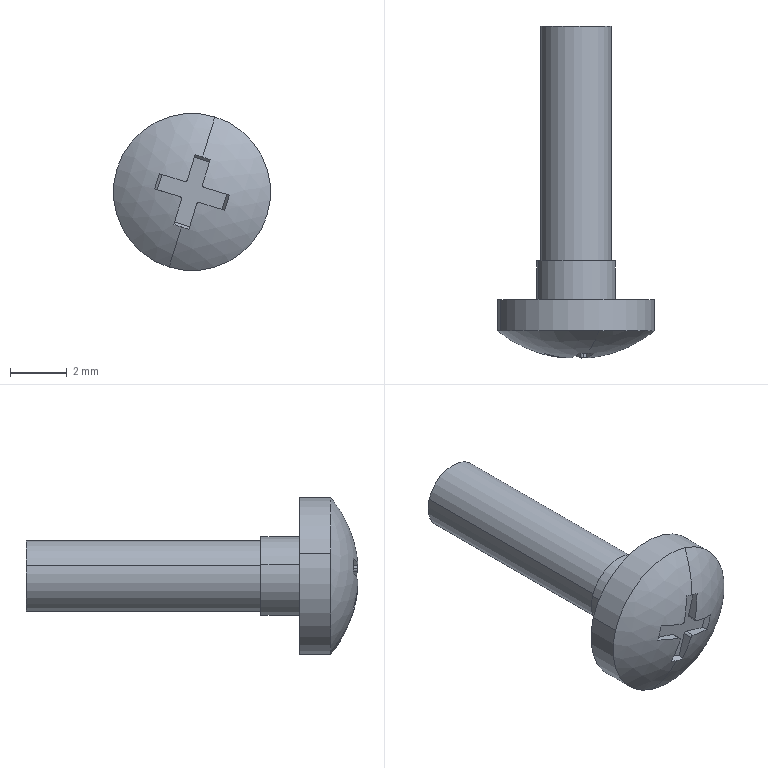Component | SolidWorks | cross recessed small pan head screws gb1-1 | 1 solid | 28 faces | box 5.56 x 11.73 x 5.56 mm | volume 87 mm3 | plane 16 | cylinder 10 | sphere 2 | commonest cylinder face diameters 0.167 x4 2.5 x2 5.556 x2 2.778 x2
STEP:
#1=COLOUR_RGB('',0.7922,0.8196,0.9333);
#2=FILL_AREA_STYLE_COLOUR('',#1);
#3=FILL_AREA_STYLE('',(#2));
#4=SURFACE_STYLE_FILL_AREA(#3);
#5=SURFACE_SIDE_STYLE('',(#4));
#6=SURFACE_STYLE_USAGE(.BOTH.,#5);
#7=PRESENTATION_STYLE_ASSIGNMENT((#6));
#8=CARTESIAN_POINT('',(-0.7465,0.7087,2.14));
#9=VERTEX_POINT('',#8);
#10=CARTESIAN_POINT('',(-0.6523,0.7087,2.112));
#11=VERTEX_POINT('',#10);
#12=CARTESIAN_POINT('',(-0.6994,0.7087,2.126));
#13=DIRECTION('',(0.,1.,0.));
#14=DIRECTION('',(-0.9565,0.,0.2917));
#15=AXIS2_PLACEMENT_3D('',#12,#13,#14);
#16=CIRCLE('',#15,0.04921);
#17=EDGE_CURVE('',#9,#11,#16,.T.);
#18=ORIENTED_EDGE('',*,*,#17,.T.);
#19=CARTESIAN_POINT('',(-0.6523,1.035,2.112));
#20=VERTEX_POINT('',#19);
#21=CARTESIAN_POINT('',(-0.6523,0.7087,2.112));
#22=DIRECTION('',(0.,1.,0.));
#23=VECTOR('',#22,39.37);
#24=LINE('',#21,#23);
#25=EDGE_CURVE('',#11,#20,#24,.T.);
#26=ORIENTED_EDGE('',*,*,#25,.T.);
#27=CARTESIAN_POINT('',(-0.7465,1.035,2.14));
#28=VERTEX_POINT('',#27);
#29=CARTESIAN_POINT('',(-0.6994,1.035,2.126));
#30=DIRECTION('',(0.,1.,0.));
#31=DIRECTION('',(-0.9565,0.,0.2917));
#32=AXIS2_PLACEMENT_3D('',#29,#30,#31);
#33=CIRCLE('',#32,0.04921);
#34=EDGE_CURVE('',#28,#20,#33,.T.);
#35=ORIENTED_EDGE('',*,*,#34,.F.);
#36=CARTESIAN_POINT('',(-0.7465,0.7087,2.14));
#37=DIRECTION('',(0.,1.,0.));
#38=VECTOR('',#37,39.37);
#39=LINE('',#36,#38);
#40=EDGE_CURVE('',#9,#28,#39,.T.);
#41=ORIENTED_EDGE('',*,*,#40,.F.);
#42=EDGE_LOOP('',(#18,#26,#35,#41));
#43=FACE_OUTER_BOUND('',#42,.T.);
#44=CARTESIAN_POINT('',(-0.6994,0.7087,2.126));
#45=DIRECTION('',(0.,1.,0.));
#46=DIRECTION('',(-0.9565,0.,0.2917));
#47=AXIS2_PLACEMENT_3D('',#44,#45,#46);
#48=CYLINDRICAL_SURFACE('',#47,0.04921);
#49=ADVANCED_FACE('',(#43),#48,.T.);
#50=CARTESIAN_POINT('',(-0.6675,0.6111,2.231));
#51=VERTEX_POINT('',#50);
#52=CARTESIAN_POINT('',(-0.5948,0.6111,2.094));
#53=VERTEX_POINT('',#52);
#54=CARTESIAN_POINT('',(-0.6994,0.6111,2.126));
#55=DIRECTION('',(0.,1.,0.));
#56=DIRECTION('',(-0.9565,0.,0.2917));
#57=AXIS2_PLACEMENT_3D('',#54,#55,#56);
#58=CIRCLE('',#57,0.1094);
#59=EDGE_CURVE('',#51,#53,#58,.T.);
#60=ORIENTED_EDGE('',*,*,#59,.T.);
#61=CARTESIAN_POINT('',(-0.5948,0.6548,2.094));
#62=VERTEX_POINT('',#61);
#63=CARTESIAN_POINT('',(-0.5948,0.6221,2.094));
#64=DIRECTION('',(0.,1.,0.));
#65=VECTOR('',#64,39.37);
#66=LINE('',#63,#65);
#67=EDGE_CURVE('',#53,#62,#66,.T.);
#68=ORIENTED_EDGE('',*,*,#67,.T.);
#69=CARTESIAN_POINT('',(-0.804,0.6548,2.158));
#70=VERTEX_POINT('',#69);
#71=CARTESIAN_POINT('',(-0.6994,0.6548,2.126));
#72=DIRECTION('',(0.,1.,0.));
#73=DIRECTION('',(-0.9565,0.,0.2917));
#74=AXIS2_PLACEMENT_3D('',#71,#72,#73);
#75=CIRCLE('',#74,0.1094);
#76=EDGE_CURVE('',#70,#62,#75,.T.);
#77=ORIENTED_EDGE('',*,*,#76,.F.);
#78=CARTESIAN_POINT('',(-0.804,0.6111,2.158));
#79=VERTEX_POINT('',#78);
#80=CARTESIAN_POINT('',(-0.804,0.6221,2.158));
#81=DIRECTION('',(0.,1.,0.));
#82=VECTOR('',#81,39.37);
#83=LINE('',#80,#82);
#84=EDGE_CURVE('',#79,#70,#83,.T.);
#85=ORIENTED_EDGE('',*,*,#84,.F.);
#86=CARTESIAN_POINT('',(-0.6994,0.6111,2.126));
#87=DIRECTION('',(0.,1.,0.));
#88=DIRECTION('',(-0.9565,0.,0.2917));
#89=AXIS2_PLACEMENT_3D('',#86,#87,#88);
#90=CIRCLE('',#89,0.1094);
#91=EDGE_CURVE('',#79,#51,#90,.T.);
#92=ORIENTED_EDGE('',*,*,#91,.T.);
#93=EDGE_LOOP('',(#60,#68,#77,#85,#92));
#94=FACE_OUTER_BOUND('',#93,.T.);
#95=CARTESIAN_POINT('',(-0.6994,0.6221,2.126));
#96=DIRECTION('',(0.,1.,0.));
#97=DIRECTION('',(-0.9565,0.,0.2917));
#98=AXIS2_PLACEMENT_3D('',#95,#96,#97);
#99=CYLINDRICAL_SURFACE('',#98,0.1094);
#100=ADVANCED_FACE('',(#94),#99,.T.);
#101=CARTESIAN_POINT('',(-0.7036,0.5806,2.074));
#102=VERTEX_POINT('',#101);
#103=CARTESIAN_POINT('',(-0.7143,0.5803,2.077));
#104=VERTEX_POINT('',#103);
#105=CARTESIAN_POINT('',(-0.6894,0.7279,2.159));
#106=DIRECTION('',(-0.2527,0.5,-0.8284));
#107=DIRECTION('',(-0.1459,-0.866,-0.4782));
#108=AXIS2_PLACEMENT_3D('',#105,#106,#107);
#109=CIRCLE('',#108,0.1704);
#110=EDGE_CURVE('',#102,#104,#109,.T.);
#111=ORIENTED_EDGE('',*,*,#110,.T.);
#112=CARTESIAN_POINT('',(-0.7313,0.6111,2.021));
#113=VERTEX_POINT('',#112);
#114=CARTESIAN_POINT('',(-0.6994,0.7477,2.126));
#115=DIRECTION('',(0.9565,-0.,-0.2917));
#116=DIRECTION('',(-0.2917,0.,-0.9565));
#117=AXIS2_PLACEMENT_3D('',#114,#115,#116);
#118=CIRCLE('',#117,0.175);
#119=EDGE_CURVE('',#104,#113,#118,.T.);
#120=ORIENTED_EDGE('',*,*,#119,.T.);
#121=CARTESIAN_POINT('',(-0.6994,0.6111,2.126));
#122=DIRECTION('',(0.,1.,0.));
#123=DIRECTION('',(-0.9565,0.,0.2917));
#124=AXIS2_PLACEMENT_3D('',#121,#122,#123);
#125=CIRCLE('',#124,0.1094);
#126=EDGE_CURVE('',#53,#113,#125,.T.);
#127=ORIENTED_EDGE('',*,*,#126,.F.);
#128=ORIENTED_EDGE('',*,*,#59,.F.);
#129=CARTESIAN_POINT('',(-0.6846,0.5803,2.175));
#130=VERTEX_POINT('',#129);
#131=CARTESIAN_POINT('',(-0.6994,0.7477,2.126));
#132=DIRECTION('',(-0.9565,0.,0.2917));
#133=DIRECTION('',(0.2917,0.,0.9565));
#134=AXIS2_PLACEMENT_3D('',#131,#132,#133);
#135=CIRCLE('',#134,0.175);
#136=EDGE_CURVE('',#130,#51,#135,.T.);
#137=ORIENTED_EDGE('',*,*,#136,.F.);
#138=CARTESIAN_POINT('',(-0.6741,0.5806,2.171));
#139=VERTEX_POINT('',#138);
#140=CARTESIAN_POINT('',(-0.7094,0.7279,2.093));
#141=DIRECTION('',(0.2527,0.5,0.8284));
#142=DIRECTION('',(-0.1459,0.866,-0.4782));
#143=AXIS2_PLACEMENT_3D('',#140,#141,#142);
#144=CIRCLE('',#143,0.1704);
#145=EDGE_CURVE('',#130,#139,#144,.T.);
#146=ORIENTED_EDGE('',*,*,#145,.T.);
#147=CARTESIAN_POINT('',(-0.6847,0.5737,2.136));
#148=VERTEX_POINT('',#147);
#149=CARTESIAN_POINT('',(-0.6889,0.7477,2.123));
#150=DIRECTION('',(0.9565,0.,-0.2917));
#151=DIRECTION('',(0.2917,0.,0.9565));
#152=AXIS2_PLACEMENT_3D('',#149,#150,#151);
#153=CIRCLE('',#152,0.1746);
#154=EDGE_CURVE('',#139,#148,#153,.T.);
#155=ORIENTED_EDGE('',*,*,#154,.T.);
#156=CARTESIAN_POINT('',(-0.6825,0.5737,2.132));
#157=VERTEX_POINT('',#156);
#158=CARTESIAN_POINT('',(-0.6847,0.5737,2.136));
#159=CARTESIAN_POINT('',(-0.6848,0.5737,2.136));
#160=CARTESIAN_POINT('',(-0.6848,0.5736,2.136));
#161=CARTESIAN_POINT('',(-0.6848,0.5736,2.135));
#162=CARTESIAN_POINT('',(-0.6848,0.5736,2.135));
#163=CARTESIAN_POINT('',(-0.6847,0.5736,2.135));
#164=CARTESIAN_POINT('',(-0.6846,0.5736,2.134));
#165=CARTESIAN_POINT('',(-0.6845,0.5736,2.134));
#166=CARTESIAN_POINT('',(-0.6843,0.5736,2.134));
#167=CARTESIAN_POINT('',(-0.684,0.5736,2.133));
#168=CARTESIAN_POINT('',(-0.6838,0.5736,2.133));
#169=CARTESIAN_POINT('',(-0.6835,0.5736,2.133));
#170=CARTESIAN_POINT('',(-0.6832,0.5736,2.133));
#171=CARTESIAN_POINT('',(-0.683,0.5736,2.133));
#172=CARTESIAN_POINT('',(-0.6827,0.5737,2.132));
#173=CARTESIAN_POINT('',(-0.6825,0.5737,2.132));
#174=B_SPLINE_CURVE_WITH_KNOTS('',3,(#158,#159,#160,#161,#162,#163,#164,#165,#166,#167,#168,#169,#170,#171,#172,#173),.UNSPECIFIED.,.F.,.F.,(4,3,3,3,3,4),(0.,0.00002794,0.00005589,0.00008373,0.0001115,0.0001303),.UNSPECIFIED.);
#175=EDGE_CURVE('',#148,#157,#174,.T.);
#176=ORIENTED_EDGE('',*,*,#175,.T.);
#177=CARTESIAN_POINT('',(-0.6477,0.5806,2.122));
#178=VERTEX_POINT('',#177);
#179=CARTESIAN_POINT('',(-0.6962,0.7477,2.137));
#180=DIRECTION('',(0.2917,0.,0.9565));
#181=DIRECTION('',(-0.9565,0.,0.2917));
#182=AXIS2_PLACEMENT_3D('',#179,#180,#181);
#183=CIRCLE('',#182,0.1746);
#184=EDGE_CURVE('',#157,#178,#183,.T.);
#185=ORIENTED_EDGE('',*,*,#184,.T.);
#186=CARTESIAN_POINT('',(-0.6542,0.5806,2.101));
#187=VERTEX_POINT('',#186);
#188=CARTESIAN_POINT('',(-0.7323,0.7279,2.136));
#189=DIRECTION('',(0.8284,0.5,-0.2527));
#190=DIRECTION('',(0.4782,-0.866,-0.1459));
#191=AXIS2_PLACEMENT_3D('',#188,#189,#190);
#192=CIRCLE('',#191,0.1704);
#193=EDGE_CURVE('',#178,#187,#192,.T.);
#194=ORIENTED_EDGE('',*,*,#193,.T.);
#195=CARTESIAN_POINT('',(-0.6889,0.5737,2.111));
#196=VERTEX_POINT('',#195);
#197=CARTESIAN_POINT('',(-0.7026,0.7477,2.115));
#198=DIRECTION('',(-0.2917,-0.,-0.9565));
#199=DIRECTION('',(0.9565,-0.,-0.2917));
#200=AXIS2_PLACEMENT_3D('',#197,#198,#199);
#201=CIRCLE('',#200,0.1746);
#202=EDGE_CURVE('',#187,#196,#201,.T.);
#203=ORIENTED_EDGE('',*,*,#202,.T.);
#204=CARTESIAN_POINT('',(-0.693,0.5737,2.109));
#205=VERTEX_POINT('',#204);
#206=CARTESIAN_POINT('',(-0.6889,0.5737,2.111));
#207=CARTESIAN_POINT('',(-0.6893,0.5737,2.111));
#208=CARTESIAN_POINT('',(-0.6897,0.5736,2.111));
#209=CARTESIAN_POINT('',(-0.69,0.5736,2.111));
#210=CARTESIAN_POINT('',(-0.6904,0.5736,2.111));
#211=CARTESIAN_POINT('',(-0.6908,0.5736,2.111));
#212=CARTESIAN_POINT('',(-0.6911,0.5736,2.111));
#213=CARTESIAN_POINT('',(-0.6914,0.5736,2.111));
#214=CARTESIAN_POINT('',(-0.6918,0.5736,2.111));
#215=CARTESIAN_POINT('',(-0.692,0.5736,2.111));
#216=CARTESIAN_POINT('',(-0.6923,0.5736,2.11));
#217=CARTESIAN_POINT('',(-0.6926,0.5736,2.11));
#218=CARTESIAN_POINT('',(-0.6927,0.5736,2.11));
#219=CARTESIAN_POINT('',(-0.6929,0.5736,2.11));
#220=CARTESIAN_POINT('',(-0.693,0.5737,2.109));
#221=CARTESIAN_POINT('',(-0.693,0.5737,2.109));
#222=B_SPLINE_CURVE_WITH_KNOTS('',3,(#206,#207,#208,#209,#210,#211,#212,#213,#214,#215,#216,#217,#218,#219,#220,#221),.UNSPECIFIED.,.F.,.F.,(4,3,3,3,3,4),(0.,0.00002794,0.00005589,0.00008373,0.0001115,0.0001303),.UNSPECIFIED.);
#223=EDGE_CURVE('',#196,#205,#222,.T.);
#224=ORIENTED_EDGE('',*,*,#223,.T.);
#225=CARTESIAN_POINT('',(-0.6889,0.7477,2.123));
#226=DIRECTION('',(0.9565,0.,-0.2917));
#227=DIRECTION('',(0.2917,0.,0.9565));
#228=AXIS2_PLACEMENT_3D('',#225,#226,#227);
#229=CIRCLE('',#228,0.1746);
#230=EDGE_CURVE('',#205,#102,#229,.T.);
#231=ORIENTED_EDGE('',*,*,#230,.T.);
#232=EDGE_LOOP('',(#111,#120,#127,#128,#137,#146,#155,#176,#185,#194,#203,#224,#231));
#233=FACE_OUTER_BOUND('',#232,.T.);
#234=CARTESIAN_POINT('',(-0.6994,0.7477,2.126));
#235=DIRECTION('',(0.9565,-0.,-0.2917));
#236=DIRECTION('',(0.2917,0.,0.9565));
#237=AXIS2_PLACEMENT_3D('',#234,#235,#236);
#238=SPHERICAL_SURFACE('',#237,0.175);
#239=ADVANCED_FACE('',(#233),#238,.T.);
#240=CARTESIAN_POINT('',(-0.7517,0.6548,2.142));
#241=VERTEX_POINT('',#240);
#242=CARTESIAN_POINT('',(-0.6471,0.6548,2.11));
#243=VERTEX_POINT('',#242);
#244=CARTESIAN_POINT('',(-0.6994,0.6548,2.126));
#245=DIRECTION('',(0.,1.,0.));
#246=DIRECTION('',(-0.9565,0.,0.2917));
#247=AXIS2_PLACEMENT_3D('',#244,#245,#246);
#248=CIRCLE('',#247,0.05468);
#249=EDGE_CURVE('',#241,#243,#248,.T.);
#250=ORIENTED_EDGE('',*,*,#249,.T.);
#251=CARTESIAN_POINT('',(-0.6471,0.7087,2.11));
#252=VERTEX_POINT('',#251);
#253=CARTESIAN_POINT('',(-0.6471,0.6221,2.11));
#254=DIRECTION('',(0.,1.,0.));
#255=VECTOR('',#254,39.37);
#256=LINE('',#253,#255);
#257=EDGE_CURVE('',#243,#252,#256,.T.);
#258=ORIENTED_EDGE('',*,*,#257,.T.);
#259=CARTESIAN_POINT('',(-0.7517,0.7087,2.142));
#260=VERTEX_POINT('',#259);
#261=CARTESIAN_POINT('',(-0.6994,0.7087,2.126));
#262=DIRECTION('',(-0.,-1.,0.));
#263=DIRECTION('',(-0.9565,0.,0.2917));
#264=AXIS2_PLACEMENT_3D('',#261,#262,#263);
#265=CIRCLE('',#264,0.05468);
#266=EDGE_CURVE('',#252,#260,#265,.T.);
#267=ORIENTED_EDGE('',*,*,#266,.T.);
#268=CARTESIAN_POINT('',(-0.7517,0.6221,2.142));
#269=DIRECTION('',(0.,1.,0.));
#270=VECTOR('',#269,39.37);
#271=LINE('',#268,#270);
#272=EDGE_CURVE('',#241,#260,#271,.T.);
#273=ORIENTED_EDGE('',*,*,#272,.F.);
#274=EDGE_LOOP('',(#250,#258,#267,#273));
#275=FACE_OUTER_BOUND('',#274,.T.);
#276=CARTESIAN_POINT('',(-0.6994,0.6221,2.126));
#277=DIRECTION('',(0.,1.,0.));
#278=DIRECTION('',(-0.9565,0.,0.2917));
#279=AXIS2_PLACEMENT_3D('',#276,#277,#278);
#280=CYLINDRICAL_SURFACE('',#279,0.05468);
#281=ADVANCED_FACE('',(#275),#280,.T.);
#282=ORIENTED_EDGE('',*,*,#257,.F.);
#283=CARTESIAN_POINT('',(-0.6994,0.6548,2.126));
#284=DIRECTION('',(0.,1.,0.));
#285=DIRECTION('',(-0.9565,0.,0.2917));
#286=AXIS2_PLACEMENT_3D('',#283,#284,#285);
#287=CIRCLE('',#286,0.05468);
#288=EDGE_CURVE('',#243,#241,#287,.T.);
#289=ORIENTED_EDGE('',*,*,#288,.T.);
#290=ORIENTED_EDGE('',*,*,#272,.T.);
#291=CARTESIAN_POINT('',(-0.6994,0.7087,2.126));
#292=DIRECTION('',(-0.,-1.,0.));
#293=DIRECTION('',(-0.9565,0.,0.2917));
#294=AXIS2_PLACEMENT_3D('',#291,#292,#293);
#295=CIRCLE('',#294,0.05468);
#296=EDGE_CURVE('',#260,#252,#295,.T.);
#297=ORIENTED_EDGE('',*,*,#296,.T.);
#298=EDGE_LOOP('',(#282,#289,#290,#297));
#299=FACE_OUTER_BOUND('',#298,.T.);
#300=CARTESIAN_POINT('',(-0.6994,0.6221,2.126));
#301=DIRECTION('',(0.,1.,0.));
#302=DIRECTION('',(-0.9565,0.,0.2917));
#303=AXIS2_PLACEMENT_3D('',#300,#301,#302);
#304=CYLINDRICAL_SURFACE('',#303,0.05468);
#305=ADVANCED_FACE('',(#299),#304,.T.);
#306=ORIENTED_EDGE('',*,*,#119,.F.);
#307=CARTESIAN_POINT('',(-0.7248,0.5806,2.081));
#308=VERTEX_POINT('',#307);
#309=CARTESIAN_POINT('',(-0.6894,0.7279,2.159));
#310=DIRECTION('',(-0.2527,0.5,-0.8284));
#311=DIRECTION('',(-0.1459,-0.866,-0.4782));
#312=AXIS2_PLACEMENT_3D('',#309,#310,#311);
#313=CIRCLE('',#312,0.1704);
#314=EDGE_CURVE('',#104,#308,#313,.T.);
#315=ORIENTED_EDGE('',*,*,#314,.T.);
#316=CARTESIAN_POINT('',(-0.7142,0.5737,2.116));
#317=VERTEX_POINT('',#316);
#318=CARTESIAN_POINT('',(-0.71,0.7477,2.129));
#319=DIRECTION('',(-0.9565,-0.,0.2917));
#320=DIRECTION('',(0.,1.,0.));
#321=AXIS2_PLACEMENT_3D('',#318,#319,#320);
#322=CIRCLE('',#321,0.1746);
#323=EDGE_CURVE('',#308,#317,#322,.T.);
#324=ORIENTED_EDGE('',*,*,#323,.T.);
#325=CARTESIAN_POINT('',(-0.7163,0.5737,2.12));
#326=VERTEX_POINT('',#325);
#327=CARTESIAN_POINT('',(-0.7142,0.5737,2.116));
#328=CARTESIAN_POINT('',(-0.7141,0.5737,2.116));
#329=CARTESIAN_POINT('',(-0.714,0.5736,2.116));
#330=CARTESIAN_POINT('',(-0.714,0.5736,2.117));
#331=CARTESIAN_POINT('',(-0.714,0.5736,2.117));
#332=CARTESIAN_POINT('',(-0.7141,0.5736,2.117));
#333=CARTESIAN_POINT('',(-0.7143,0.5736,2.118));
#334=CARTESIAN_POINT('',(-0.7144,0.5736,2.118));
#335=CARTESIAN_POINT('',(-0.7146,0.5736,2.118));
#336=CARTESIAN_POINT('',(-0.7148,0.5736,2.119));
#337=CARTESIAN_POINT('',(-0.7151,0.5736,2.119));
#338=CARTESIAN_POINT('',(-0.7153,0.5736,2.119));
#339=CARTESIAN_POINT('',(-0.7157,0.5736,2.119));
#340=CARTESIAN_POINT('',(-0.7159,0.5736,2.119));
#341=CARTESIAN_POINT('',(-0.7161,0.5737,2.12));
#342=CARTESIAN_POINT('',(-0.7163,0.5737,2.12));
#343=B_SPLINE_CURVE_WITH_KNOTS('',3,(#327,#328,#329,#330,#331,#332,#333,#334,#335,#336,#337,#338,#339,#340,#341,#342),.UNSPECIFIED.,.F.,.F.,(4,3,3,3,3,4),(0.,0.00002794,0.00005589,0.00008373,0.0001115,0.0001303),.UNSPECIFIED.);
#344=EDGE_CURVE('',#317,#326,#343,.T.);
#345=ORIENTED_EDGE('',*,*,#344,.T.);
#346=CARTESIAN_POINT('',(-0.7511,0.5806,2.13));
#347=VERTEX_POINT('',#346);
#348=CARTESIAN_POINT('',(-0.7026,0.7477,2.115));
#349=DIRECTION('',(-0.2917,0.,-0.9565));
#350=DIRECTION('',(0.9565,0.,-0.2917));
#351=AXIS2_PLACEMENT_3D('',#348,#349,#350);
#352=CIRCLE('',#351,0.1746);
#353=EDGE_CURVE('',#326,#347,#352,.T.);
#354=ORIENTED_EDGE('',*,*,#353,.T.);
#355=CARTESIAN_POINT('',(-0.7447,0.5806,2.151));
#356=VERTEX_POINT('',#355);
#357=CARTESIAN_POINT('',(-0.6666,0.7279,2.116));
#358=DIRECTION('',(-0.8284,0.5,0.2527));
#359=DIRECTION('',(0.4782,0.866,-0.1459));
#360=AXIS2_PLACEMENT_3D('',#357,#358,#359);
#361=CIRCLE('',#360,0.1704);
#362=EDGE_CURVE('',#347,#356,#361,.T.);
#363=ORIENTED_EDGE('',*,*,#362,.T.);
#364=CARTESIAN_POINT('',(-0.7099,0.5737,2.141));
#365=VERTEX_POINT('',#364);
#366=CARTESIAN_POINT('',(-0.6962,0.7477,2.137));
#367=DIRECTION('',(0.2917,0.,0.9565));
#368=DIRECTION('',(-0.9565,-0.,0.2917));
#369=AXIS2_PLACEMENT_3D('',#366,#367,#368);
#370=CIRCLE('',#369,0.1746);
#371=EDGE_CURVE('',#356,#365,#370,.T.);
#372=ORIENTED_EDGE('',*,*,#371,.T.);
#373=CARTESIAN_POINT('',(-0.7058,0.5737,2.143));
#374=VERTEX_POINT('',#373);
#375=CARTESIAN_POINT('',(-0.7099,0.5737,2.141));
#376=CARTESIAN_POINT('',(-0.7096,0.5737,2.141));
#377=CARTESIAN_POINT('',(-0.7092,0.5736,2.141));
#378=CARTESIAN_POINT('',(-0.7088,0.5736,2.141));
#379=CARTESIAN_POINT('',(-0.7084,0.5736,2.141));
#380=CARTESIAN_POINT('',(-0.7081,0.5736,2.141));
#381=CARTESIAN_POINT('',(-0.7077,0.5736,2.141));
#382=CARTESIAN_POINT('',(-0.7074,0.5736,2.141));
#383=CARTESIAN_POINT('',(-0.7071,0.5736,2.141));
#384=CARTESIAN_POINT('',(-0.7068,0.5736,2.141));
#385=CARTESIAN_POINT('',(-0.7065,0.5736,2.142));
#386=CARTESIAN_POINT('',(-0.7063,0.5736,2.142));
#387=CARTESIAN_POINT('',(-0.7061,0.5736,2.142));
#388=CARTESIAN_POINT('',(-0.706,0.5736,2.142));
#389=CARTESIAN_POINT('',(-0.7059,0.5737,2.143));
#390=CARTESIAN_POINT('',(-0.7058,0.5737,2.143));
#391=B_SPLINE_CURVE_WITH_KNOTS('',3,(#375,#376,#377,#378,#379,#380,#381,#382,#383,#384,#385,#386,#387,#388,#389,#390),.UNSPECIFIED.,.F.,.F.,(4,3,3,3,3,4),(0.,0.00002794,0.00005589,0.00008373,0.0001115,0.0001303),.UNSPECIFIED.);
#392=EDGE_CURVE('',#365,#374,#391,.T.);
#393=ORIENTED_EDGE('',*,*,#392,.T.);
#394=CARTESIAN_POINT('',(-0.6952,0.5806,2.178));
#395=VERTEX_POINT('',#394);
#396=CARTESIAN_POINT('',(-0.71,0.7477,2.129));
#397=DIRECTION('',(-0.9565,-0.,0.2917));
#398=DIRECTION('',(0.,1.,0.));
#399=AXIS2_PLACEMENT_3D('',#396,#397,#398);
#400=CIRCLE('',#399,0.1746);
#401=EDGE_CURVE('',#374,#395,#400,.T.);
#402=ORIENTED_EDGE('',*,*,#401,.T.);
#403=CARTESIAN_POINT('',(-0.7094,0.7279,2.093));
#404=DIRECTION('',(0.2527,0.5,0.8284));
#405=DIRECTION('',(-0.1459,0.866,-0.4782));
#406=AXIS2_PLACEMENT_3D('',#403,#404,#405);
#407=CIRCLE('',#406,0.1704);
#408=EDGE_CURVE('',#395,#130,#407,.T.);
#409=ORIENTED_EDGE('',*,*,#408,.T.);
#410=ORIENTED_EDGE('',*,*,#136,.T.);
#411=ORIENTED_EDGE('',*,*,#91,.F.);
#412=CARTESIAN_POINT('',(-0.6994,0.6111,2.126));
#413=DIRECTION('',(0.,1.,0.));
#414=DIRECTION('',(-0.9565,0.,0.2917));
#415=AXIS2_PLACEMENT_3D('',#412,#413,#414);
#416=CIRCLE('',#415,0.1094);
#417=EDGE_CURVE('',#113,#79,#416,.T.);
#418=ORIENTED_EDGE('',*,*,#417,.F.);
#419=EDGE_LOOP('',(#306,#315,#324,#345,#354,#363,#372,#393,#402,#409,#410,#411,#418));
#420=FACE_OUTER_BOUND('',#419,.T.);
#421=CARTESIAN_POINT('',(-0.6994,0.7477,2.126));
#422=DIRECTION('',(0.9565,-0.,-0.2917));
#423=DIRECTION('',(0.2917,0.,0.9565));
#424=AXIS2_PLACEMENT_3D('',#421,#422,#423);
#425=SPHERICAL_SURFACE('',#424,0.175);
#426=ADVANCED_FACE('',(#420),#425,.T.);
#427=ORIENTED_EDGE('',*,*,#76,.T.);
#428=CARTESIAN_POINT('',(-0.6994,0.6548,2.126));
#429=DIRECTION('',(0.,1.,0.));
#430=DIRECTION('',(-0.9565,0.,0.2917));
#431=AXIS2_PLACEMENT_3D('',#428,#429,#430);
#432=CIRCLE('',#431,0.1094);
#433=EDGE_CURVE('',#62,#70,#432,.T.);
#434=ORIENTED_EDGE('',*,*,#433,.T.);
#435=EDGE_LOOP('',(#427,#434));
#436=FACE_OUTER_BOUND('',#435,.T.);
#437=ORIENTED_EDGE('',*,*,#249,.F.);
#438=ORIENTED_EDGE('',*,*,#288,.F.);
#439=EDGE_LOOP('',(#437,#438));
#440=FACE_BOUND('',#439,.T.);
#441=CARTESIAN_POINT('',(-0.6816,0.6548,2.185));
#442=DIRECTION('',(0.,1.,0.));
#443=DIRECTION('',(-0.9565,-0.,0.2917));
#444=AXIS2_PLACEMENT_3D('',#441,#442,#443);
#445=PLANE('',#444);
#446=ADVANCED_FACE('',(#436,#440),#445,.T.);
#447=ORIENTED_EDGE('',*,*,#67,.F.);
#448=ORIENTED_EDGE('',*,*,#126,.T.);
#449=ORIENTED_EDGE('',*,*,#417,.T.);
#450=ORIENTED_EDGE('',*,*,#84,.T.);
#451=ORIENTED_EDGE('',*,*,#433,.F.);
#452=EDGE_LOOP('',(#447,#448,#449,#450,#451));
#453=FACE_OUTER_BOUND('',#452,.T.);
#454=CARTESIAN_POINT('',(-0.6994,0.6221,2.126));
#455=DIRECTION('',(0.,1.,0.));
#456=DIRECTION('',(-0.9565,0.,0.2917));
#457=AXIS2_PLACEMENT_3D('',#454,#455,#456);
#458=CYLINDRICAL_SURFACE('',#457,0.1094);
#459=ADVANCED_FACE('',(#453),#458,.T.);
#460=ORIENTED_EDGE('',*,*,#184,.F.);
#461=CARTESIAN_POINT('',(-0.6825,0.587,2.132));
#462=VERTEX_POINT('',#461);
#463=CARTESIAN_POINT('',(-0.6825,0.587,2.132));
#464=DIRECTION('',(0.,1.,0.));
#465=VECTOR('',#464,39.37);
#466=LINE('',#463,#465);
#467=EDGE_CURVE('',#157,#462,#466,.T.);
#468=ORIENTED_EDGE('',*,*,#467,.T.);
#469=CARTESIAN_POINT('',(-0.6512,0.587,2.123));
#470=VERTEX_POINT('',#469);
#471=CARTESIAN_POINT('',(-0.6856,0.587,2.133));
#472=DIRECTION('',(0.9565,0.,-0.2917));
#473=VECTOR('',#472,39.37);
#474=LINE('',#471,#473);
#475=EDGE_CURVE('',#462,#470,#474,.T.);
#476=ORIENTED_EDGE('',*,*,#475,.T.);
#477=CARTESIAN_POINT('',(-0.6434,0.5727,2.12));
#478=DIRECTION('',(0.4782,-0.866,-0.1459));
#479=VECTOR('',#478,39.37);
#480=LINE('',#477,#479);
#481=EDGE_CURVE('',#470,#178,#480,.T.);
#482=ORIENTED_EDGE('',*,*,#481,.T.);
#483=EDGE_LOOP('',(#460,#468,#476,#482));
#484=FACE_OUTER_BOUND('',#483,.T.);
#485=CARTESIAN_POINT('',(-0.6856,0.587,2.133));
#486=DIRECTION('',(-0.2917,-0.,-0.9565));
#487=DIRECTION('',(-0.9565,-0.,0.2917));
#488=AXIS2_PLACEMENT_3D('',#485,#486,#487);
#489=PLANE('',#488);
#490=ADVANCED_FACE('',(#484),#489,.T.);
#491=ORIENTED_EDGE('',*,*,#481,.F.);
#492=CARTESIAN_POINT('',(-0.6577,0.587,2.102));
#493=VERTEX_POINT('',#492);
#494=CARTESIAN_POINT('',(-0.6544,0.587,2.112));
#495=DIRECTION('',(-0.2917,0.,-0.9565));
#496=VECTOR('',#495,39.37);
#497=LINE('',#494,#496);
#498=EDGE_CURVE('',#470,#493,#497,.T.);
#499=ORIENTED_EDGE('',*,*,#498,.T.);
#500=CARTESIAN_POINT('',(-0.6663,0.6025,2.104));
#501=DIRECTION('',(0.4782,-0.866,-0.1459));
#502=VECTOR('',#501,39.37);
#503=LINE('',#500,#502);
#504=EDGE_CURVE('',#493,#187,#503,.T.);
#505=ORIENTED_EDGE('',*,*,#504,.T.);
#506=ORIENTED_EDGE('',*,*,#193,.F.);
#507=EDGE_LOOP('',(#491,#499,#505,#506));
#508=FACE_OUTER_BOUND('',#507,.T.);
#509=CARTESIAN_POINT('',(-0.6466,0.5727,2.11));
#510=DIRECTION('',(-0.8284,-0.5,0.2527));
#511=DIRECTION('',(0.4782,-0.866,-0.1459));
#512=AXIS2_PLACEMENT_3D('',#509,#510,#511);
#513=PLANE('',#512);
#514=ADVANCED_FACE('',(#508),#513,.T.);
#515=CARTESIAN_POINT('',(-0.6889,0.587,2.111));
#516=VERTEX_POINT('',#515);
#517=CARTESIAN_POINT('',(-0.6921,0.587,2.112));
#518=DIRECTION('',(-0.9565,-0.,0.2917));
#519=VECTOR('',#518,39.37);
#520=LINE('',#517,#519);
#521=EDGE_CURVE('',#493,#516,#520,.T.);
#522=ORIENTED_EDGE('',*,*,#521,.T.);
#523=CARTESIAN_POINT('',(-0.6889,0.587,2.111));
#524=DIRECTION('',(-0.,-1.,0.));
#525=VECTOR('',#524,39.37);
#526=LINE('',#523,#525);
#527=EDGE_CURVE('',#516,#196,#526,.T.);
#528=ORIENTED_EDGE('',*,*,#527,.T.);
#529=ORIENTED_EDGE('',*,*,#202,.F.);
#530=ORIENTED_EDGE('',*,*,#504,.F.);
#531=EDGE_LOOP('',(#522,#528,#529,#530));
#532=FACE_OUTER_BOUND('',#531,.T.);
#533=CARTESIAN_POINT('',(-0.6921,0.587,2.112));
#534=DIRECTION('',(0.2917,0.,0.9565));
#535=DIRECTION('',(0.9565,0.,-0.2917));
#536=AXIS2_PLACEMENT_3D('',#533,#534,#535);
#537=PLANE('',#536);
#538=ADVANCED_FACE('',(#532),#537,.T.);
#539=ORIENTED_EDGE('',*,*,#230,.F.);
#540=CARTESIAN_POINT('',(-0.693,0.587,2.109));
#541=VERTEX_POINT('',#540);
#542=CARTESIAN_POINT('',(-0.693,0.587,2.109));
#543=DIRECTION('',(0.,1.,0.));
#544=VECTOR('',#543,39.37);
#545=LINE('',#542,#544);
#546=EDGE_CURVE('',#205,#541,#545,.T.);
#547=ORIENTED_EDGE('',*,*,#546,.T.);
#548=CARTESIAN_POINT('',(-0.7026,0.587,2.078));
#549=VERTEX_POINT('',#548);
#550=CARTESIAN_POINT('',(-0.6921,0.587,2.112));
#551=DIRECTION('',(-0.2917,-0.,-0.9565));
#552=VECTOR('',#551,39.37);
#553=LINE('',#550,#552);
#554=EDGE_CURVE('',#541,#549,#553,.T.);
#555=ORIENTED_EDGE('',*,*,#554,.T.);
#556=CARTESIAN_POINT('',(-0.705,0.5727,2.07));
#557=DIRECTION('',(-0.1459,-0.866,-0.4782));
#558=VECTOR('',#557,39.37);
#559=LINE('',#556,#558);
#560=EDGE_CURVE('',#549,#102,#559,.T.);
#561=ORIENTED_EDGE('',*,*,#560,.T.);
#562=EDGE_LOOP('',(#539,#547,#555,#561));
#563=FACE_OUTER_BOUND('',#562,.T.);
#564=CARTESIAN_POINT('',(-0.6921,0.587,2.112));
#565=DIRECTION('',(-0.9565,-0.,0.2917));
#566=DIRECTION('',(0.2917,0.,0.9565));
#567=AXIS2_PLACEMENT_3D('',#564,#565,#566);
#568=PLANE('',#567);
#569=ADVANCED_FACE('',(#563),#568,.T.);
#570=ORIENTED_EDGE('',*,*,#560,.F.);
#571=CARTESIAN_POINT('',(-0.7237,0.587,2.084));
#572=VERTEX_POINT('',#571);
#573=CARTESIAN_POINT('',(-0.7131,0.587,2.081));
#574=DIRECTION('',(-0.9565,-0.,0.2917));
#575=VECTOR('',#574,39.37);
#576=LINE('',#573,#575);
#577=EDGE_CURVE('',#549,#572,#576,.T.);
#578=ORIENTED_EDGE('',*,*,#577,.T.);
#579=CARTESIAN_POINT('',(-0.7211,0.6025,2.093));
#580=DIRECTION('',(-0.1459,-0.866,-0.4782));
#581=VECTOR('',#580,39.37);
#582=LINE('',#579,#581);
#583=EDGE_CURVE('',#572,#308,#582,.T.);
#584=ORIENTED_EDGE('',*,*,#583,.T.);
#585=ORIENTED_EDGE('',*,*,#314,.F.);
#586=ORIENTED_EDGE('',*,*,#110,.F.);
#587=EDGE_LOOP('',(#570,#578,#584,#585,#586));
#588=FACE_OUTER_BOUND('',#587,.T.);
#589=CARTESIAN_POINT('',(-0.7155,0.5727,2.073));
#590=DIRECTION('',(0.2527,-0.5,0.8284));
#591=DIRECTION('',(-0.1459,-0.866,-0.4782));
#592=AXIS2_PLACEMENT_3D('',#589,#590,#591);
#593=PLANE('',#592);
#594=ADVANCED_FACE('',(#588),#593,.T.);
#595=CARTESIAN_POINT('',(-0.7142,0.587,2.116));
#596=VERTEX_POINT('',#595);
#597=CARTESIAN_POINT('',(-0.7132,0.587,2.119));
#598=DIRECTION('',(0.2917,0.,0.9565));
#599=VECTOR('',#598,39.37);
#600=LINE('',#597,#599);
#601=EDGE_CURVE('',#572,#596,#600,.T.);
#602=ORIENTED_EDGE('',*,*,#601,.T.);
#603=CARTESIAN_POINT('',(-0.7142,0.587,2.116));
#604=DIRECTION('',(-0.,-1.,0.));
#605=VECTOR('',#604,39.37);
#606=LINE('',#603,#605);
#607=EDGE_CURVE('',#596,#317,#606,.T.);
#608=ORIENTED_EDGE('',*,*,#607,.T.);
#609=ORIENTED_EDGE('',*,*,#323,.F.);
#610=ORIENTED_EDGE('',*,*,#583,.F.);
#611=EDGE_LOOP('',(#602,#608,#609,#610));
#612=FACE_OUTER_BOUND('',#611,.T.);
#613=CARTESIAN_POINT('',(-0.7132,0.587,2.119));
#614=DIRECTION('',(0.9565,-0.,-0.2917));
#615=DIRECTION('',(0.,1.,0.));
#616=AXIS2_PLACEMENT_3D('',#613,#614,#615);
#617=PLANE('',#616);
#618=ADVANCED_FACE('',(#612),#617,.T.);
#619=ORIENTED_EDGE('',*,*,#353,.F.);
#620=CARTESIAN_POINT('',(-0.7163,0.587,2.12));
#621=VERTEX_POINT('',#620);
#622=CARTESIAN_POINT('',(-0.7163,0.587,2.12));
#623=DIRECTION('',(0.,1.,0.));
#624=VECTOR('',#623,39.37);
#625=LINE('',#622,#624);
#626=EDGE_CURVE('',#326,#621,#625,.T.);
#627=ORIENTED_EDGE('',*,*,#626,.T.);
#628=CARTESIAN_POINT('',(-0.7476,0.587,2.129));
#629=VERTEX_POINT('',#628);
#630=CARTESIAN_POINT('',(-0.7132,0.587,2.119));
#631=DIRECTION('',(-0.9565,-0.,0.2917));
#632=VECTOR('',#631,39.37);
#633=LINE('',#630,#632);
#634=EDGE_CURVE('',#621,#629,#633,.T.);
#635=ORIENTED_EDGE('',*,*,#634,.T.);
#636=CARTESIAN_POINT('',(-0.7555,0.5727,2.132));
#637=DIRECTION('',(-0.4782,-0.866,0.1459));
#638=VECTOR('',#637,39.37);
#639=LINE('',#636,#638);
#640=EDGE_CURVE('',#629,#347,#639,.T.);
#641=ORIENTED_EDGE('',*,*,#640,.T.);
#642=EDGE_LOOP('',(#619,#627,#635,#641));
#643=FACE_OUTER_BOUND('',#642,.T.);
#644=CARTESIAN_POINT('',(-0.7132,0.587,2.119));
#645=DIRECTION('',(0.2917,0.,0.9565));
#646=DIRECTION('',(0.9565,0.,-0.2917));
#647=AXIS2_PLACEMENT_3D('',#644,#645,#646);
#648=PLANE('',#647);
#649=ADVANCED_FACE('',(#643),#648,.T.);
#650=ORIENTED_EDGE('',*,*,#640,.F.);
#651=CARTESIAN_POINT('',(-0.7412,0.587,2.15));
#652=VERTEX_POINT('',#651);
#653=CARTESIAN_POINT('',(-0.7444,0.587,2.14));
#654=DIRECTION('',(0.2917,0.,0.9565));
#655=VECTOR('',#654,39.37);
#656=LINE('',#653,#655);
#657=EDGE_CURVE('',#629,#652,#656,.T.);
#658=ORIENTED_EDGE('',*,*,#657,.T.);
#659=CARTESIAN_POINT('',(-0.7326,0.6025,2.148));
#660=DIRECTION('',(-0.4782,-0.866,0.1459));
#661=VECTOR('',#660,39.37);
#662=LINE('',#659,#661);
#663=EDGE_CURVE('',#652,#356,#662,.T.);
#664=ORIENTED_EDGE('',*,*,#663,.T.);
#665=ORIENTED_EDGE('',*,*,#362,.F.);
#666=EDGE_LOOP('',(#650,#658,#664,#665));
#667=FACE_OUTER_BOUND('',#666,.T.);
#668=CARTESIAN_POINT('',(-0.7522,0.5727,2.142));
#669=DIRECTION('',(0.8284,-0.5,-0.2527));
#670=DIRECTION('',(0.4782,0.866,-0.1459));
#671=AXIS2_PLACEMENT_3D('',#668,#669,#670);
#672=PLANE('',#671);
#673=ADVANCED_FACE('',(#667),#672,.T.);
#674=CARTESIAN_POINT('',(-0.7099,0.587,2.141));
#675=VERTEX_POINT('',#674);
#676=CARTESIAN_POINT('',(-0.7068,0.587,2.14));
#677=DIRECTION('',(0.9565,0.,-0.2917));
#678=VECTOR('',#677,39.37);
#679=LINE('',#676,#678);
#680=EDGE_CURVE('',#652,#675,#679,.T.);
#681=ORIENTED_EDGE('',*,*,#680,.T.);
#682=CARTESIAN_POINT('',(-0.7099,0.587,2.141));
#683=DIRECTION('',(-0.,-1.,0.));
#684=VECTOR('',#683,39.37);
#685=LINE('',#682,#684);
#686=EDGE_CURVE('',#675,#365,#685,.T.);
#687=ORIENTED_EDGE('',*,*,#686,.T.);
#688=ORIENTED_EDGE('',*,*,#371,.F.);
#689=ORIENTED_EDGE('',*,*,#663,.F.);
#690=EDGE_LOOP('',(#681,#687,#688,#689));
#691=FACE_OUTER_BOUND('',#690,.T.);
#692=CARTESIAN_POINT('',(-0.7068,0.587,2.14));
#693=DIRECTION('',(-0.2917,0.,-0.9565));
#694=DIRECTION('',(-0.9565,-0.,0.2917));
#695=AXIS2_PLACEMENT_3D('',#692,#693,#694);
#696=PLANE('',#695);
#697=ADVANCED_FACE('',(#691),#696,.T.);
#698=ORIENTED_EDGE('',*,*,#401,.F.);
#699=CARTESIAN_POINT('',(-0.7058,0.587,2.143));
#700=VERTEX_POINT('',#699);
#701=CARTESIAN_POINT('',(-0.7058,0.587,2.143));
#702=DIRECTION('',(0.,1.,0.));
#703=VECTOR('',#702,39.37);
#704=LINE('',#701,#703);
#705=EDGE_CURVE('',#374,#700,#704,.T.);
#706=ORIENTED_EDGE('',*,*,#705,.T.);
#707=CARTESIAN_POINT('',(-0.6963,0.587,2.174));
#708=VERTEX_POINT('',#707);
#709=CARTESIAN_POINT('',(-0.7068,0.587,2.14));
#710=DIRECTION('',(0.2917,0.,0.9565));
#711=VECTOR('',#710,39.37);
#712=LINE('',#709,#711);
#713=EDGE_CURVE('',#700,#708,#712,.T.);
#714=ORIENTED_EDGE('',*,*,#713,.T.);
#715=CARTESIAN_POINT('',(-0.6939,0.5727,2.182));
#716=DIRECTION('',(0.1459,-0.866,0.4782));
#717=VECTOR('',#716,39.37);
#718=LINE('',#715,#717);
#719=EDGE_CURVE('',#708,#395,#718,.T.);
#720=ORIENTED_EDGE('',*,*,#719,.T.);
#721=EDGE_LOOP('',(#698,#706,#714,#720));
#722=FACE_OUTER_BOUND('',#721,.T.);
#723=CARTESIAN_POINT('',(-0.7068,0.587,2.14));
#724=DIRECTION('',(0.9565,-0.,-0.2917));
#725=DIRECTION('',(0.,1.,0.));
#726=AXIS2_PLACEMENT_3D('',#723,#724,#725);
#727=PLANE('',#726);
#728=ADVANCED_FACE('',(#722),#727,.T.);
#729=ORIENTED_EDGE('',*,*,#719,.F.);
#730=CARTESIAN_POINT('',(-0.6751,0.587,2.168));
#731=VERTEX_POINT('',#730);
#732=CARTESIAN_POINT('',(-0.6857,0.587,2.171));
#733=DIRECTION('',(0.9565,0.,-0.2917));
#734=VECTOR('',#733,39.37);
#735=LINE('',#732,#734);
#736=EDGE_CURVE('',#708,#731,#735,.T.);
#737=ORIENTED_EDGE('',*,*,#736,.T.);
#738=CARTESIAN_POINT('',(-0.6778,0.6025,2.159));
#739=DIRECTION('',(0.1459,-0.866,0.4782));
#740=VECTOR('',#739,39.37);
#741=LINE('',#738,#740);
#742=EDGE_CURVE('',#731,#139,#741,.T.);
#743=ORIENTED_EDGE('',*,*,#742,.T.);
#744=ORIENTED_EDGE('',*,*,#145,.F.);
#745=ORIENTED_EDGE('',*,*,#408,.F.);
#746=EDGE_LOOP('',(#729,#737,#743,#744,#745));
#747=FACE_OUTER_BOUND('',#746,.T.);
#748=CARTESIAN_POINT('',(-0.6833,0.5727,2.179));
#749=DIRECTION('',(-0.2527,-0.5,-0.8284));
#750=DIRECTION('',(-0.1459,0.866,-0.4782));
#751=AXIS2_PLACEMENT_3D('',#748,#749,#750);
#752=PLANE('',#751);
#753=ADVANCED_FACE('',(#747),#752,.T.);
#754=CARTESIAN_POINT('',(-0.6847,0.587,2.136));
#755=VERTEX_POINT('',#754);
#756=CARTESIAN_POINT('',(-0.6856,0.587,2.133));
#757=DIRECTION('',(-0.2917,-0.,-0.9565));
#758=VECTOR('',#757,39.37);
#759=LINE('',#756,#758);
#760=EDGE_CURVE('',#731,#755,#759,.T.);
#761=ORIENTED_EDGE('',*,*,#760,.T.);
#762=CARTESIAN_POINT('',(-0.6847,0.587,2.136));
#763=DIRECTION('',(-0.,-1.,0.));
#764=VECTOR('',#763,39.37);
#765=LINE('',#762,#764);
#766=EDGE_CURVE('',#755,#148,#765,.T.);
#767=ORIENTED_EDGE('',*,*,#766,.T.);
#768=ORIENTED_EDGE('',*,*,#154,.F.);
#769=ORIENTED_EDGE('',*,*,#742,.F.);
#770=EDGE_LOOP('',(#761,#767,#768,#769));
#771=FACE_OUTER_BOUND('',#770,.T.);
#772=CARTESIAN_POINT('',(-0.6856,0.587,2.133));
#773=DIRECTION('',(-0.9565,-0.,0.2917));
#774=DIRECTION('',(0.2917,0.,0.9565));
#775=AXIS2_PLACEMENT_3D('',#772,#773,#774);
#776=PLANE('',#775);
#777=ADVANCED_FACE('',(#771),#776,.T.);
#778=ORIENTED_EDGE('',*,*,#475,.F.);
#779=CARTESIAN_POINT('',(-0.6815,0.587,2.136));
#780=DIRECTION('',(0.,1.,0.));
#781=DIRECTION('',(-0.9565,0.,0.2917));
#782=AXIS2_PLACEMENT_3D('',#779,#780,#781);
#783=CIRCLE('',#782,0.003281);
#784=EDGE_CURVE('',#462,#755,#783,.T.);
#785=ORIENTED_EDGE('',*,*,#784,.T.);
#786=ORIENTED_EDGE('',*,*,#760,.F.);
#787=ORIENTED_EDGE('',*,*,#736,.F.);
#788=ORIENTED_EDGE('',*,*,#713,.F.);
#789=CARTESIAN_POINT('',(-0.7089,0.587,2.144));
#790=DIRECTION('',(0.,1.,0.));
#791=DIRECTION('',(-0.9565,0.,0.2917));
#792=AXIS2_PLACEMENT_3D('',#789,#790,#791);
#793=CIRCLE('',#792,0.003281);
#794=EDGE_CURVE('',#700,#675,#793,.T.);
#795=ORIENTED_EDGE('',*,*,#794,.T.);
#796=ORIENTED_EDGE('',*,*,#680,.F.);
#797=ORIENTED_EDGE('',*,*,#657,.F.);
#798=ORIENTED_EDGE('',*,*,#634,.F.);
#799=CARTESIAN_POINT('',(-0.7173,0.587,2.116));
#800=DIRECTION('',(0.,1.,0.));
#801=DIRECTION('',(-0.9565,0.,0.2917));
#802=AXIS2_PLACEMENT_3D('',#799,#800,#801);
#803=CIRCLE('',#802,0.003281);
#804=EDGE_CURVE('',#621,#596,#803,.T.);
#805=ORIENTED_EDGE('',*,*,#804,.T.);
#806=ORIENTED_EDGE('',*,*,#601,.F.);
#807=ORIENTED_EDGE('',*,*,#577,.F.);
#808=ORIENTED_EDGE('',*,*,#554,.F.);
#809=CARTESIAN_POINT('',(-0.6899,0.587,2.108));
#810=DIRECTION('',(0.,1.,0.));
#811=DIRECTION('',(-0.9565,0.,0.2917));
#812=AXIS2_PLACEMENT_3D('',#809,#810,#811);
#813=CIRCLE('',#812,0.003281);
#814=EDGE_CURVE('',#541,#516,#813,.T.);
#815=ORIENTED_EDGE('',*,*,#814,.T.);
#816=ORIENTED_EDGE('',*,*,#521,.F.);
#817=ORIENTED_EDGE('',*,*,#498,.F.);
#818=EDGE_LOOP('',(#778,#785,#786,#787,#788,#795,#796,#797,#798,#805,#806,#807,#808,#815,#816,#817));
#819=FACE_OUTER_BOUND('',#818,.T.);
#820=CARTESIAN_POINT('',(-0.6856,0.587,2.133));
#821=DIRECTION('',(0.,1.,0.));
#822=DIRECTION('',(-0.9565,-0.,0.2917));
#823=AXIS2_PLACEMENT_3D('',#820,#821,#822);
#824=PLANE('',#823);
#825=ADVANCED_FACE('',(#819),#824,.F.);
#826=ORIENTED_EDGE('',*,*,#814,.F.);
#827=ORIENTED_EDGE('',*,*,#546,.F.);
#828=ORIENTED_EDGE('',*,*,#223,.F.);
#829=ORIENTED_EDGE('',*,*,#527,.F.);
#830=EDGE_LOOP('',(#826,#827,#828,#829));
#831=FACE_OUTER_BOUND('',#830,.T.);
#832=CARTESIAN_POINT('',(-0.6899,0.587,2.108));
#833=DIRECTION('',(-0.,-1.,0.));
#834=DIRECTION('',(0.9565,0.,-0.2917));
#835=AXIS2_PLACEMENT_3D('',#832,#833,#834);
#836=CYLINDRICAL_SURFACE('',#835,0.003281);
#837=ADVANCED_FACE('',(#831),#836,.T.);
#838=ORIENTED_EDGE('',*,*,#804,.F.);
#839=ORIENTED_EDGE('',*,*,#626,.F.);
#840=ORIENTED_EDGE('',*,*,#344,.F.);
#841=ORIENTED_EDGE('',*,*,#607,.F.);
#842=EDGE_LOOP('',(#838,#839,#840,#841));
#843=FACE_OUTER_BOUND('',#842,.T.);
#844=CARTESIAN_POINT('',(-0.7173,0.587,2.116));
#845=DIRECTION('',(-0.,-1.,0.));
#846=DIRECTION('',(0.9565,0.,-0.2917));
#847=AXIS2_PLACEMENT_3D('',#844,#845,#846);
#848=CYLINDRICAL_SURFACE('',#847,0.003281);
#849=ADVANCED_FACE('',(#843),#848,.T.);
#850=ORIENTED_EDGE('',*,*,#784,.F.);
#851=ORIENTED_EDGE('',*,*,#467,.F.);
#852=ORIENTED_EDGE('',*,*,#175,.F.);
#853=ORIENTED_EDGE('',*,*,#766,.F.);
#854=EDGE_LOOP('',(#850,#851,#852,#853));
#855=FACE_OUTER_BOUND('',#854,.T.);
#856=CARTESIAN_POINT('',(-0.6815,0.587,2.136));
#857=DIRECTION('',(-0.,-1.,0.));
#858=DIRECTION('',(0.9565,0.,-0.2917));
#859=AXIS2_PLACEMENT_3D('',#856,#857,#858);
#860=CYLINDRICAL_SURFACE('',#859,0.003281);
#861=ADVANCED_FACE('',(#855),#860,.T.);
#862=ORIENTED_EDGE('',*,*,#794,.F.);
#863=ORIENTED_EDGE('',*,*,#705,.F.);
#864=ORIENTED_EDGE('',*,*,#392,.F.);
#865=ORIENTED_EDGE('',*,*,#686,.F.);
#866=EDGE_LOOP('',(#862,#863,#864,#865));
#867=FACE_OUTER_BOUND('',#866,.T.);
#868=CARTESIAN_POINT('',(-0.7089,0.587,2.144));
#869=DIRECTION('',(-0.,-1.,0.));
#870=DIRECTION('',(0.9565,0.,-0.2917));
#871=AXIS2_PLACEMENT_3D('',#868,#869,#870);
#872=CYLINDRICAL_SURFACE('',#871,0.003281);
#873=ADVANCED_FACE('',(#867),#872,.T.);
#874=ORIENTED_EDGE('',*,*,#296,.F.);
#875=ORIENTED_EDGE('',*,*,#266,.F.);
#876=EDGE_LOOP('',(#874,#875));
#877=FACE_OUTER_BOUND('',#876,.T.);
#878=ORIENTED_EDGE('',*,*,#17,.F.);
#879=CARTESIAN_POINT('',(-0.6994,0.7087,2.126));
#880=DIRECTION('',(0.,1.,0.));
#881=DIRECTION('',(-0.9565,0.,0.2917));
#882=AXIS2_PLACEMENT_3D('',#879,#880,#881);
#883=CIRCLE('',#882,0.04921);
#884=EDGE_CURVE('',#11,#9,#883,.T.);
#885=ORIENTED_EDGE('',*,*,#884,.F.);
#886=EDGE_LOOP('',(#878,#885));
#887=FACE_BOUND('',#886,.T.);
#888=CARTESIAN_POINT('',(-0.6994,0.7087,2.126));
#889=DIRECTION('',(0.,1.,0.));
#890=DIRECTION('',(-0.9565,-0.,0.2917));
#891=AXIS2_PLACEMENT_3D('',#888,#889,#890);
#892=PLANE('',#891);
#893=ADVANCED_FACE('',(#877,#887),#892,.T.);
#894=ORIENTED_EDGE('',*,*,#25,.F.);
#895=ORIENTED_EDGE('',*,*,#884,.T.);
#896=ORIENTED_EDGE('',*,*,#40,.T.);
#897=CARTESIAN_POINT('',(-0.6994,1.035,2.126));
#898=DIRECTION('',(0.,1.,0.));
#899=DIRECTION('',(-0.9565,0.,0.2917));
#900=AXIS2_PLACEMENT_3D('',#897,#898,#899);
#901=CIRCLE('',#900,0.04921);
#902=EDGE_CURVE('',#20,#28,#901,.T.);
#903=ORIENTED_EDGE('',*,*,#902,.F.);
#904=EDGE_LOOP('',(#894,#895,#896,#903));
#905=FACE_OUTER_BOUND('',#904,.T.);
#906=CARTESIAN_POINT('',(-0.6994,0.7087,2.126));
#907=DIRECTION('',(0.,1.,0.));
#908=DIRECTION('',(-0.9565,0.,0.2917));
#909=AXIS2_PLACEMENT_3D('',#906,#907,#908);
#910=CYLINDRICAL_SURFACE('',#909,0.04921);
#911=ADVANCED_FACE('',(#905),#910,.T.);
#912=ORIENTED_EDGE('',*,*,#34,.T.);
#913=ORIENTED_EDGE('',*,*,#902,.T.);
#914=EDGE_LOOP('',(#912,#913));
#915=FACE_OUTER_BOUND('',#914,.T.);
#916=CARTESIAN_POINT('',(-0.6994,1.035,2.126));
#917=DIRECTION('',(0.,1.,0.));
#918=DIRECTION('',(-0.9565,-0.,0.2917));
#919=AXIS2_PLACEMENT_3D('',#916,#917,#918);
#920=PLANE('',#919);
#921=ADVANCED_FACE('',(#915),#920,.T.);
#922=CLOSED_SHELL('',(#49,#100,#239,#281,#305,#426,#446,#459,#490,#514,#538,#569,#594,#618,#649,#673,#697,#728,#753,#777,#825,#837,#849,#861,#873,#893,#911,#921));
#923=MANIFOLD_SOLID_BREP('',#922);
#924=STYLED_ITEM('',(#7),#923);
#925=(LENGTH_UNIT()NAMED_UNIT(*)SI_UNIT($,.METRE.));
#926=LENGTH_MEASURE_WITH_UNIT(LENGTH_MEASURE(0.0254),#925);
#927=DIMENSIONAL_EXPONENTS(1.,0.,0.,0.,0.,0.,0.);
#928=(CONVERSION_BASED_UNIT('',#926)LENGTH_UNIT()NAMED_UNIT(#927));
#929=UNCERTAINTY_MEASURE_WITH_UNIT(LENGTH_MEASURE(0.00001),#928,'','');
#930=(NAMED_UNIT(*)PLANE_ANGLE_UNIT()SI_UNIT($,.RADIAN.));
#931=(NAMED_UNIT(*)SI_UNIT($,.STERADIAN.)SOLID_ANGLE_UNIT());
#932=(GEOMETRIC_REPRESENTATION_CONTEXT(3)GLOBAL_UNCERTAINTY_ASSIGNED_CONTEXT((#929))GLOBAL_UNIT_ASSIGNED_CONTEXT((#928,#930,#931))REPRESENTATION_CONTEXT('',''));
#933=MECHANICAL_DESIGN_GEOMETRIC_PRESENTATION_REPRESENTATION('',(#924),#932);
#934=PRESENTATION_LAYER_ASSIGNMENT('','',(#924));
#935=CARTESIAN_POINT('',(0.,0.,0.));
#936=DIRECTION('',(0.,0.,1.));
#937=DIRECTION('',(1.,0.,0.));
#938=AXIS2_PLACEMENT_3D('',#935,#936,#937);
#939=(LENGTH_UNIT()NAMED_UNIT(*)SI_UNIT($,.METRE.));
#940=LENGTH_MEASURE_WITH_UNIT(LENGTH_MEASURE(0.0254),#939);
#941=DIMENSIONAL_EXPONENTS(1.,0.,0.,0.,0.,0.,0.);
#942=(CONVERSION_BASED_UNIT('',#940)LENGTH_UNIT()NAMED_UNIT(#941));
#943=UNCERTAINTY_MEASURE_WITH_UNIT(LENGTH_MEASURE(0.00001),#942,'','');
#944=(NAMED_UNIT(*)PLANE_ANGLE_UNIT()SI_UNIT($,.RADIAN.));
#945=(NAMED_UNIT(*)SI_UNIT($,.STERADIAN.)SOLID_ANGLE_UNIT());
#946=(GEOMETRIC_REPRESENTATION_CONTEXT(3)GLOBAL_UNCERTAINTY_ASSIGNED_CONTEXT((#943))GLOBAL_UNIT_ASSIGNED_CONTEXT((#942,#944,#945))REPRESENTATION_CONTEXT('',''));
#947=ADVANCED_BREP_SHAPE_REPRESENTATION('',(#923,#938),#946);